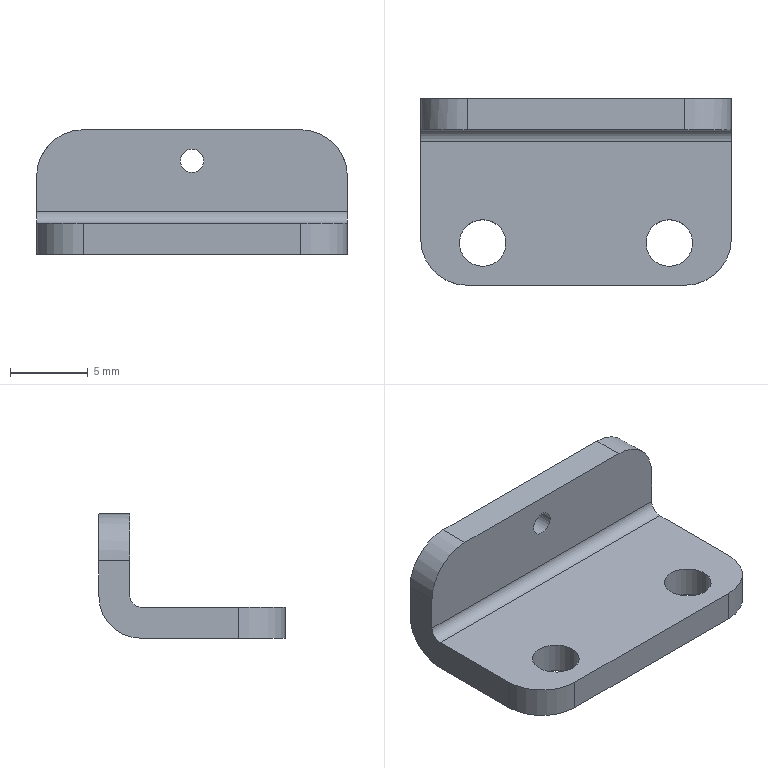Component | NX | BASE-MOUNTING-BRACKET_2 | 1 solid | 17 faces | volume 643 mm3 | cylinder 9 | plane 8 | commonest cylinder face diameters 6 x4 1.5 x2 3 x2 5.5 x1